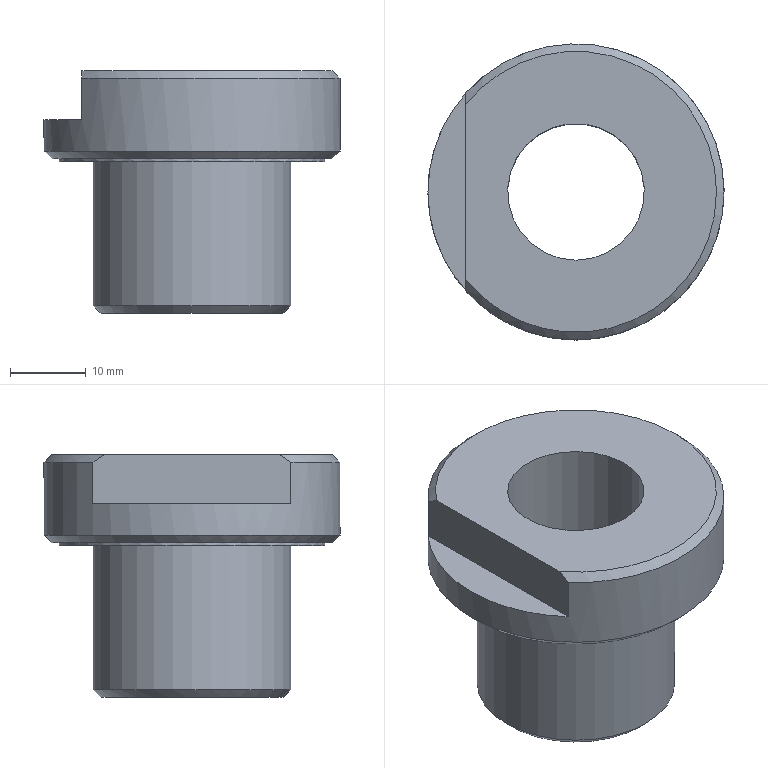Component | NX | REPL_DRILL_BUSH | 1 solid | 14 faces | box 39 x 39 x 32 mm | volume 15961 mm3 | plane 6 | cylinder 4 | cone 4 | commonest cylinder face diameters 26 x1 35 x1 39 x1 18 x1
STEP:
#1=CARTESIAN_POINT('',(0.,0.,0.));
#2=DIRECTION('',(0.,0.,1.));
#3=DIRECTION('',(1.,0.,0.));
#4=AXIS2_PLACEMENT_3D('',#1,#2,#3);
#5=CARTESIAN_POINT('',(32.,-10.,-160.));
#6=VERTEX_POINT('',#5);
#7=CARTESIAN_POINT('',(32.,-0.,-160.));
#8=DIRECTION('',(0.,0.,1.));
#9=DIRECTION('',(0.,-1.,0.));
#10=AXIS2_PLACEMENT_3D('',#7,#8,#9);
#11=CIRCLE('',#10,10.);
#12=CARTESIAN_POINT('',(32.,-0.,-160.));
#13=DIRECTION('',(0.,0.,-1.));
#14=DIRECTION('',(0.,-1.,0.));
#15=AXIS2_PLACEMENT_3D('',#12,#13,#14);
#16=PLANE('',#15);
#17=CARTESIAN_POINT('',(10.,0.));
#18=CARTESIAN_POINT('',(10.,-17.321));
#19=CARTESIAN_POINT('',(-5.,-8.66));
#20=CARTESIAN_POINT('',(-20.,-0.));
#21=CARTESIAN_POINT('',(-5.,8.66));
#22=CARTESIAN_POINT('',(10.,17.321));
#23=CARTESIAN_POINT('',(10.,0.));
#24=(BOUNDED_CURVE()B_SPLINE_CURVE(2,(#17,#18,#19,#20,#21,#22,#23),.UNSPECIFIED.,.T.,.F.)B_SPLINE_CURVE_WITH_KNOTS((1,2,2,2,2,1),(-2.094,0.,2.094,4.189,6.283,8.378),.UNSPECIFIED.)CURVE()GEOMETRIC_REPRESENTATION_ITEM()RATIONAL_B_SPLINE_CURVE((1.,0.5,1.,0.5,1.,0.5,1.))REPRESENTATION_ITEM(''));
#25=(GEOMETRIC_REPRESENTATION_CONTEXT(2)PARAMETRIC_REPRESENTATION_CONTEXT()REPRESENTATION_CONTEXT('',''));
#26=DEFINITIONAL_REPRESENTATION('',(#24),#25);
#27=PCURVE('',#16,#26);
#28=CARTESIAN_POINT('',(32.,-0.,-159.));
#29=DIRECTION('',(0.,0.,-1.));
#30=DIRECTION('',(0.,-1.,0.));
#31=AXIS2_PLACEMENT_3D('',#28,#29,#30);
#32=CONICAL_SURFACE('',#31,9.,0.7854);
#33=CARTESIAN_POINT('',(6.283,1.));
#34=DIRECTION('',(-1.,0.));
#35=VECTOR('',#34,1.);
#36=LINE('',#33,#35);
#37=(GEOMETRIC_REPRESENTATION_CONTEXT(2)PARAMETRIC_REPRESENTATION_CONTEXT()REPRESENTATION_CONTEXT('',''));
#38=DEFINITIONAL_REPRESENTATION('',(#36),#37);
#39=PCURVE('',#32,#38);
#40=SURFACE_CURVE('',#11,(#27,#39),.PCURVE_S1.);
#41=EDGE_CURVE('',#6,#6,#40,.T.);
#42=ORIENTED_EDGE('',*,*,#41,.T.);
#43=EDGE_LOOP('',(#42));
#44=FACE_BOUND('',#43,.T.);
#45=CARTESIAN_POINT('',(32.,-12.,-160.));
#46=VERTEX_POINT('',#45);
#47=CARTESIAN_POINT('',(32.,-0.,-160.));
#48=DIRECTION('',(0.,0.,-1.));
#49=DIRECTION('',(0.,-1.,0.));
#50=AXIS2_PLACEMENT_3D('',#47,#48,#49);
#51=CIRCLE('',#50,12.);
#52=CARTESIAN_POINT('',(0.,0.));
#53=DIRECTION('',(1.,0.));
#54=AXIS2_PLACEMENT_2D('',#52,#53);
#55=CIRCLE('',#54,12.);
#56=(GEOMETRIC_REPRESENTATION_CONTEXT(2)PARAMETRIC_REPRESENTATION_CONTEXT()REPRESENTATION_CONTEXT('',''));
#57=DEFINITIONAL_REPRESENTATION('',(#55),#56);
#58=PCURVE('',#16,#57);
#59=CARTESIAN_POINT('',(32.,-0.,-159.));
#60=DIRECTION('',(0.,0.,1.));
#61=DIRECTION('',(0.,1.,0.));
#62=AXIS2_PLACEMENT_3D('',#59,#60,#61);
#63=CONICAL_SURFACE('',#62,13.,0.7854);
#64=CARTESIAN_POINT('',(9.425,-1.));
#65=DIRECTION('',(-1.,0.));
#66=VECTOR('',#65,1.);
#67=LINE('',#64,#66);
#68=(GEOMETRIC_REPRESENTATION_CONTEXT(2)PARAMETRIC_REPRESENTATION_CONTEXT()REPRESENTATION_CONTEXT('',''));
#69=DEFINITIONAL_REPRESENTATION('',(#67),#68);
#70=PCURVE('',#63,#69);
#71=SURFACE_CURVE('',#51,(#58,#70),.PCURVE_S1.);
#72=EDGE_CURVE('',#46,#46,#71,.T.);
#73=ORIENTED_EDGE('',*,*,#72,.T.);
#74=EDGE_LOOP('',(#73));
#75=FACE_BOUND('',#74,.T.);
#76=ADVANCED_FACE('',(#44,#75),#16,.T.);
#77=CARTESIAN_POINT('',(32.,-13.,-159.));
#78=VERTEX_POINT('',#77);
#79=CARTESIAN_POINT('',(32.,-0.,-159.));
#80=DIRECTION('',(0.,0.,1.));
#81=DIRECTION('',(0.,-1.,0.));
#82=AXIS2_PLACEMENT_3D('',#79,#80,#81);
#83=CIRCLE('',#82,13.);
#84=CARTESIAN_POINT('',(32.,-0.,-160.));
#85=DIRECTION('',(0.,0.,1.));
#86=DIRECTION('',(0.,1.,0.));
#87=AXIS2_PLACEMENT_3D('',#84,#85,#86);
#88=CYLINDRICAL_SURFACE('',#87,13.);
#89=CARTESIAN_POINT('',(3.142,1.));
#90=DIRECTION('',(1.,0.));
#91=VECTOR('',#90,1.);
#92=LINE('',#89,#91);
#93=(GEOMETRIC_REPRESENTATION_CONTEXT(2)PARAMETRIC_REPRESENTATION_CONTEXT()REPRESENTATION_CONTEXT('',''));
#94=DEFINITIONAL_REPRESENTATION('',(#92),#93);
#95=PCURVE('',#88,#94);
#96=CARTESIAN_POINT('',(3.142,0.));
#97=DIRECTION('',(1.,0.));
#98=VECTOR('',#97,1.);
#99=LINE('',#96,#98);
#100=(GEOMETRIC_REPRESENTATION_CONTEXT(2)PARAMETRIC_REPRESENTATION_CONTEXT()REPRESENTATION_CONTEXT('',''));
#101=DEFINITIONAL_REPRESENTATION('',(#99),#100);
#102=PCURVE('',#63,#101);
#103=SURFACE_CURVE('',#83,(#95,#102),.PCURVE_S1.);
#104=EDGE_CURVE('',#78,#78,#103,.T.);
#105=ORIENTED_EDGE('',*,*,#104,.T.);
#106=CARTESIAN_POINT('',(32.,-13.,-140.));
#107=VERTEX_POINT('',#106);
#108=CARTESIAN_POINT('',(32.,-13.,-159.));
#109=CARTESIAN_POINT('',(32.,-13.,-140.));
#110=B_SPLINE_CURVE_WITH_KNOTS('',1,(#108,#109),.UNSPECIFIED.,.F.,.F.,(2,2),(1.,20.),.PIECEWISE_BEZIER_KNOTS.);
#111=CARTESIAN_POINT('',(9.425,0.));
#112=DIRECTION('',(0.,1.));
#113=VECTOR('',#112,1.);
#114=LINE('',#111,#113);
#115=(GEOMETRIC_REPRESENTATION_CONTEXT(2)PARAMETRIC_REPRESENTATION_CONTEXT()REPRESENTATION_CONTEXT('',''));
#116=DEFINITIONAL_REPRESENTATION('',(#114),#115);
#117=PCURVE('',#88,#116);
#118=CARTESIAN_POINT('',(3.142,0.));
#119=DIRECTION('',(0.,1.));
#120=VECTOR('',#119,1.);
#121=LINE('',#118,#120);
#122=(GEOMETRIC_REPRESENTATION_CONTEXT(2)PARAMETRIC_REPRESENTATION_CONTEXT()REPRESENTATION_CONTEXT('',''));
#123=DEFINITIONAL_REPRESENTATION('',(#121),#122);
#124=PCURVE('',#88,#123);
#125=SEAM_CURVE('',#110,(#117,#124),.PCURVE_S1.);
#126=EDGE_CURVE('',#78,#107,#125,.T.);
#127=ORIENTED_EDGE('',*,*,#126,.T.);
#128=CARTESIAN_POINT('',(32.,-0.,-140.));
#129=DIRECTION('',(0.,0.,1.));
#130=DIRECTION('',(0.,-1.,0.));
#131=AXIS2_PLACEMENT_3D('',#128,#129,#130);
#132=CIRCLE('',#131,13.);
#133=CARTESIAN_POINT('',(3.142,20.));
#134=DIRECTION('',(1.,0.));
#135=VECTOR('',#134,1.);
#136=LINE('',#133,#135);
#137=(GEOMETRIC_REPRESENTATION_CONTEXT(2)PARAMETRIC_REPRESENTATION_CONTEXT()REPRESENTATION_CONTEXT('',''));
#138=DEFINITIONAL_REPRESENTATION('',(#136),#137);
#139=PCURVE('',#88,#138);
#140=CARTESIAN_POINT('',(32.,-0.,-140.));
#141=DIRECTION('',(0.,0.,-1.));
#142=DIRECTION('',(0.,-1.,0.));
#143=AXIS2_PLACEMENT_3D('',#140,#141,#142);
#144=PLANE('',#143);
#145=CARTESIAN_POINT('',(13.,0.));
#146=CARTESIAN_POINT('',(13.,-22.517));
#147=CARTESIAN_POINT('',(-6.5,-11.258));
#148=CARTESIAN_POINT('',(-26.,-0.));
#149=CARTESIAN_POINT('',(-6.5,11.258));
#150=CARTESIAN_POINT('',(13.,22.517));
#151=CARTESIAN_POINT('',(13.,0.));
#152=(BOUNDED_CURVE()B_SPLINE_CURVE(2,(#145,#146,#147,#148,#149,#150,#151),.UNSPECIFIED.,.T.,.F.)B_SPLINE_CURVE_WITH_KNOTS((1,2,2,2,2,1),(-2.094,0.,2.094,4.189,6.283,8.378),.UNSPECIFIED.)CURVE()GEOMETRIC_REPRESENTATION_ITEM()RATIONAL_B_SPLINE_CURVE((1.,0.5,1.,0.5,1.,0.5,1.))REPRESENTATION_ITEM(''));
#153=(GEOMETRIC_REPRESENTATION_CONTEXT(2)PARAMETRIC_REPRESENTATION_CONTEXT()REPRESENTATION_CONTEXT('',''));
#154=DEFINITIONAL_REPRESENTATION('',(#152),#153);
#155=PCURVE('',#144,#154);
#156=SURFACE_CURVE('',#132,(#139,#155),.PCURVE_S1.);
#157=EDGE_CURVE('',#107,#107,#156,.T.);
#158=ORIENTED_EDGE('',*,*,#157,.F.);
#159=ORIENTED_EDGE('',*,*,#126,.F.);
#160=EDGE_LOOP('',(#105,#127,#158,#159));
#161=FACE_BOUND('',#160,.T.);
#162=ADVANCED_FACE('',(#161),#88,.T.);
#163=ORIENTED_EDGE('',*,*,#157,.T.);
#164=EDGE_LOOP('',(#163));
#165=FACE_BOUND('',#164,.T.);
#166=CARTESIAN_POINT('',(32.,17.5,-140.));
#167=VERTEX_POINT('',#166);
#168=CARTESIAN_POINT('',(32.,-0.,-140.));
#169=DIRECTION('',(0.,0.,1.));
#170=DIRECTION('',(0.,1.,0.));
#171=AXIS2_PLACEMENT_3D('',#168,#169,#170);
#172=CIRCLE('',#171,17.5);
#173=CARTESIAN_POINT('',(-17.5,0.));
#174=CARTESIAN_POINT('',(-17.5,30.311));
#175=CARTESIAN_POINT('',(8.75,15.155));
#176=CARTESIAN_POINT('',(35.,0.));
#177=CARTESIAN_POINT('',(8.75,-15.155));
#178=CARTESIAN_POINT('',(-17.5,-30.311));
#179=CARTESIAN_POINT('',(-17.5,0.));
#180=(BOUNDED_CURVE()B_SPLINE_CURVE(2,(#173,#174,#175,#176,#177,#178,#179),.UNSPECIFIED.,.T.,.F.)B_SPLINE_CURVE_WITH_KNOTS((1,2,2,2,2,1),(-2.094,0.,2.094,4.189,6.283,8.378),.UNSPECIFIED.)CURVE()GEOMETRIC_REPRESENTATION_ITEM()RATIONAL_B_SPLINE_CURVE((1.,0.5,1.,0.5,1.,0.5,1.))REPRESENTATION_ITEM(''));
#181=(GEOMETRIC_REPRESENTATION_CONTEXT(2)PARAMETRIC_REPRESENTATION_CONTEXT()REPRESENTATION_CONTEXT('',''));
#182=DEFINITIONAL_REPRESENTATION('',(#180),#181);
#183=PCURVE('',#144,#182);
#184=CARTESIAN_POINT('',(32.,-0.,-140.));
#185=DIRECTION('',(0.,0.,1.));
#186=DIRECTION('',(0.,1.,0.));
#187=AXIS2_PLACEMENT_3D('',#184,#185,#186);
#188=CYLINDRICAL_SURFACE('',#187,17.5);
#189=CARTESIAN_POINT('',(0.,0.));
#190=DIRECTION('',(1.,0.));
#191=VECTOR('',#190,1.);
#192=LINE('',#189,#191);
#193=(GEOMETRIC_REPRESENTATION_CONTEXT(2)PARAMETRIC_REPRESENTATION_CONTEXT()REPRESENTATION_CONTEXT('',''));
#194=DEFINITIONAL_REPRESENTATION('',(#192),#193);
#195=PCURVE('',#188,#194);
#196=SURFACE_CURVE('',#172,(#183,#195),.PCURVE_S1.);
#197=EDGE_CURVE('',#167,#167,#196,.T.);
#198=ORIENTED_EDGE('',*,*,#197,.F.);
#199=EDGE_LOOP('',(#198));
#200=FACE_BOUND('',#199,.T.);
#201=ADVANCED_FACE('',(#165,#200),#144,.T.);
#202=CARTESIAN_POINT('',(32.,17.5,-139.6));
#203=VERTEX_POINT('',#202);
#204=CARTESIAN_POINT('',(32.,-17.5,-139.6));
#205=VERTEX_POINT('',#204);
#206=CARTESIAN_POINT('',(32.,-0.,-139.6));
#207=DIRECTION('',(0.,0.,1.));
#208=DIRECTION('',(0.,-1.,0.));
#209=AXIS2_PLACEMENT_3D('',#206,#207,#208);
#210=CIRCLE('',#209,17.5);
#211=CARTESIAN_POINT('',(-3.142,0.4));
#212=DIRECTION('',(1.,0.));
#213=VECTOR('',#212,1.);
#214=LINE('',#211,#213);
#215=(GEOMETRIC_REPRESENTATION_CONTEXT(2)PARAMETRIC_REPRESENTATION_CONTEXT()REPRESENTATION_CONTEXT('',''));
#216=DEFINITIONAL_REPRESENTATION('',(#214),#215);
#217=PCURVE('',#188,#216);
#218=CARTESIAN_POINT('',(32.,-0.,-139.6));
#219=DIRECTION('',(0.,0.,-1.));
#220=DIRECTION('',(0.,-1.,0.));
#221=AXIS2_PLACEMENT_3D('',#218,#219,#220);
#222=PLANE('',#221);
#223=CARTESIAN_POINT('',(17.5,0.));
#224=CARTESIAN_POINT('',(17.5,-30.311));
#225=CARTESIAN_POINT('',(-8.75,-15.155));
#226=CARTESIAN_POINT('',(-35.,-0.));
#227=CARTESIAN_POINT('',(-8.75,15.155));
#228=CARTESIAN_POINT('',(17.5,30.311));
#229=CARTESIAN_POINT('',(17.5,0.));
#230=(BOUNDED_CURVE()B_SPLINE_CURVE(2,(#223,#224,#225,#226,#227,#228,#229),.UNSPECIFIED.,.T.,.F.)B_SPLINE_CURVE_WITH_KNOTS((1,2,2,2,2,1),(-2.094,0.,2.094,4.189,6.283,8.378),.UNSPECIFIED.)CURVE()GEOMETRIC_REPRESENTATION_ITEM()RATIONAL_B_SPLINE_CURVE((1.,0.5,1.,0.5,1.,0.5,1.))REPRESENTATION_ITEM(''));
#231=(GEOMETRIC_REPRESENTATION_CONTEXT(2)PARAMETRIC_REPRESENTATION_CONTEXT()REPRESENTATION_CONTEXT('',''));
#232=DEFINITIONAL_REPRESENTATION('',(#230),#231);
#233=PCURVE('',#222,#232);
#234=SURFACE_CURVE('',#210,(#217,#233),.PCURVE_S1.);
#235=EDGE_CURVE('',#203,#205,#234,.T.);
#236=ORIENTED_EDGE('',*,*,#235,.F.);
#237=CARTESIAN_POINT('',(32.,17.5,-140.));
#238=CARTESIAN_POINT('',(32.,17.5,-139.6));
#239=B_SPLINE_CURVE_WITH_KNOTS('',1,(#237,#238),.UNSPECIFIED.,.F.,.F.,(2,2),(0.,0.4),.PIECEWISE_BEZIER_KNOTS.);
#240=CARTESIAN_POINT('',(0.,0.));
#241=DIRECTION('',(0.,1.));
#242=VECTOR('',#241,1.);
#243=LINE('',#240,#242);
#244=(GEOMETRIC_REPRESENTATION_CONTEXT(2)PARAMETRIC_REPRESENTATION_CONTEXT()REPRESENTATION_CONTEXT('',''));
#245=DEFINITIONAL_REPRESENTATION('',(#243),#244);
#246=PCURVE('',#188,#245);
#247=CARTESIAN_POINT('',(6.283,0.));
#248=DIRECTION('',(0.,1.));
#249=VECTOR('',#248,1.);
#250=LINE('',#247,#249);
#251=(GEOMETRIC_REPRESENTATION_CONTEXT(2)PARAMETRIC_REPRESENTATION_CONTEXT()REPRESENTATION_CONTEXT('',''));
#252=DEFINITIONAL_REPRESENTATION('',(#250),#251);
#253=PCURVE('',#188,#252);
#254=SEAM_CURVE('',#239,(#246,#253),.PCURVE_S1.);
#255=EDGE_CURVE('',#167,#203,#254,.T.);
#256=ORIENTED_EDGE('',*,*,#255,.F.);
#257=ORIENTED_EDGE('',*,*,#197,.T.);
#258=ORIENTED_EDGE('',*,*,#255,.T.);
#259=CARTESIAN_POINT('',(32.,-0.,-139.6));
#260=DIRECTION('',(0.,0.,1.));
#261=DIRECTION('',(0.,-1.,0.));
#262=AXIS2_PLACEMENT_3D('',#259,#260,#261);
#263=CIRCLE('',#262,17.5);
#264=CARTESIAN_POINT('',(3.142,0.4));
#265=DIRECTION('',(1.,0.));
#266=VECTOR('',#265,1.);
#267=LINE('',#264,#266);
#268=(GEOMETRIC_REPRESENTATION_CONTEXT(2)PARAMETRIC_REPRESENTATION_CONTEXT()REPRESENTATION_CONTEXT('',''));
#269=DEFINITIONAL_REPRESENTATION('',(#267),#268);
#270=PCURVE('',#188,#269);
#271=CARTESIAN_POINT('',(17.5,0.));
#272=CARTESIAN_POINT('',(17.5,-30.311));
#273=CARTESIAN_POINT('',(-8.75,-15.155));
#274=CARTESIAN_POINT('',(-35.,-0.));
#275=CARTESIAN_POINT('',(-8.75,15.155));
#276=CARTESIAN_POINT('',(17.5,30.311));
#277=CARTESIAN_POINT('',(17.5,0.));
#278=(BOUNDED_CURVE()B_SPLINE_CURVE(2,(#271,#272,#273,#274,#275,#276,#277),.UNSPECIFIED.,.T.,.F.)B_SPLINE_CURVE_WITH_KNOTS((1,2,2,2,2,1),(-2.094,0.,2.094,4.189,6.283,8.378),.UNSPECIFIED.)CURVE()GEOMETRIC_REPRESENTATION_ITEM()RATIONAL_B_SPLINE_CURVE((1.,0.5,1.,0.5,1.,0.5,1.))REPRESENTATION_ITEM(''));
#279=(GEOMETRIC_REPRESENTATION_CONTEXT(2)PARAMETRIC_REPRESENTATION_CONTEXT()REPRESENTATION_CONTEXT('',''));
#280=DEFINITIONAL_REPRESENTATION('',(#278),#279);
#281=PCURVE('',#222,#280);
#282=SURFACE_CURVE('',#263,(#270,#281),.PCURVE_S1.);
#283=EDGE_CURVE('',#205,#203,#282,.T.);
#284=ORIENTED_EDGE('',*,*,#283,.F.);
#285=EDGE_LOOP('',(#236,#256,#257,#258,#284));
#286=FACE_BOUND('',#285,.T.);
#287=ADVANCED_FACE('',(#286),#188,.T.);
#288=CARTESIAN_POINT('',(32.,-9.,-128.));
#289=VERTEX_POINT('',#288);
#290=CARTESIAN_POINT('',(32.,-0.,-128.));
#291=DIRECTION('',(0.,0.,-1.));
#292=DIRECTION('',(0.,-1.,0.));
#293=AXIS2_PLACEMENT_3D('',#290,#291,#292);
#294=CIRCLE('',#293,9.);
#295=CARTESIAN_POINT('',(32.,-0.,-128.));
#296=DIRECTION('',(0.,0.,1.));
#297=DIRECTION('',(0.,1.,0.));
#298=AXIS2_PLACEMENT_3D('',#295,#296,#297);
#299=PLANE('',#298);
#300=CARTESIAN_POINT('',(-9.,0.));
#301=CARTESIAN_POINT('',(-9.,15.588));
#302=CARTESIAN_POINT('',(4.5,7.794));
#303=CARTESIAN_POINT('',(18.,0.));
#304=CARTESIAN_POINT('',(4.5,-7.794));
#305=CARTESIAN_POINT('',(-9.,-15.588));
#306=CARTESIAN_POINT('',(-9.,0.));
#307=(BOUNDED_CURVE()B_SPLINE_CURVE(2,(#300,#301,#302,#303,#304,#305,#306),.UNSPECIFIED.,.T.,.F.)B_SPLINE_CURVE_WITH_KNOTS((1,2,2,2,2,1),(-2.094,0.,2.094,4.189,6.283,8.378),.UNSPECIFIED.)CURVE()GEOMETRIC_REPRESENTATION_ITEM()RATIONAL_B_SPLINE_CURVE((1.,0.5,1.,0.5,1.,0.5,1.))REPRESENTATION_ITEM(''));
#308=(GEOMETRIC_REPRESENTATION_CONTEXT(2)PARAMETRIC_REPRESENTATION_CONTEXT()REPRESENTATION_CONTEXT('',''));
#309=DEFINITIONAL_REPRESENTATION('',(#307),#308);
#310=PCURVE('',#299,#309);
#311=CARTESIAN_POINT('',(32.,-0.,-128.));
#312=DIRECTION('',(0.,0.,-1.));
#313=DIRECTION('',(0.,-1.,0.));
#314=AXIS2_PLACEMENT_3D('',#311,#312,#313);
#315=CYLINDRICAL_SURFACE('',#314,9.);
#316=CARTESIAN_POINT('',(0.,0.));
#317=DIRECTION('',(1.,0.));
#318=VECTOR('',#317,1.);
#319=LINE('',#316,#318);
#320=(GEOMETRIC_REPRESENTATION_CONTEXT(2)PARAMETRIC_REPRESENTATION_CONTEXT()REPRESENTATION_CONTEXT('',''));
#321=DEFINITIONAL_REPRESENTATION('',(#319),#320);
#322=PCURVE('',#315,#321);
#323=SURFACE_CURVE('',#294,(#310,#322),.PCURVE_S1.);
#324=EDGE_CURVE('',#289,#289,#323,.T.);
#325=ORIENTED_EDGE('',*,*,#324,.T.);
#326=EDGE_LOOP('',(#325));
#327=FACE_BOUND('',#326,.T.);
#328=CARTESIAN_POINT('',(17.5,-11.489,-128.));
#329=VERTEX_POINT('',#328);
#330=CARTESIAN_POINT('',(17.5,11.489,-128.));
#331=VERTEX_POINT('',#330);
#332=CARTESIAN_POINT('',(17.5,-34.5,-128.));
#333=DIRECTION('',(-0.,1.,0.));
#334=VECTOR('',#333,1.);
#335=LINE('',#332,#334);
#336=CARTESIAN_POINT('',(-34.5,14.5));
#337=DIRECTION('',(1.,0.));
#338=VECTOR('',#337,1.);
#339=LINE('',#336,#338);
#340=(GEOMETRIC_REPRESENTATION_CONTEXT(2)PARAMETRIC_REPRESENTATION_CONTEXT()REPRESENTATION_CONTEXT('',''));
#341=DEFINITIONAL_REPRESENTATION('',(#339),#340);
#342=PCURVE('',#299,#341);
#343=CARTESIAN_POINT('',(17.5,-34.5,-134.5));
#344=DIRECTION('',(1.,0.,0.));
#345=DIRECTION('',(-0.,1.,0.));
#346=AXIS2_PLACEMENT_3D('',#343,#344,#345);
#347=PLANE('',#346);
#348=CARTESIAN_POINT('',(0.,6.5));
#349=DIRECTION('',(1.,0.));
#350=VECTOR('',#349,1.);
#351=LINE('',#348,#350);
#352=(GEOMETRIC_REPRESENTATION_CONTEXT(2)PARAMETRIC_REPRESENTATION_CONTEXT()REPRESENTATION_CONTEXT('',''));
#353=DEFINITIONAL_REPRESENTATION('',(#351),#352);
#354=PCURVE('',#347,#353);
#355=SURFACE_CURVE('',#335,(#342,#354),.PCURVE_S1.);
#356=EDGE_CURVE('',#329,#331,#355,.T.);
#357=ORIENTED_EDGE('',*,*,#356,.F.);
#358=CARTESIAN_POINT('',(32.,-0.,-128.));
#359=DIRECTION('',(0.,0.,1.));
#360=DIRECTION('',(0.,1.,0.));
#361=AXIS2_PLACEMENT_3D('',#358,#359,#360);
#362=CIRCLE('',#361,18.5);
#363=CARTESIAN_POINT('',(0.,0.));
#364=DIRECTION('',(1.,0.));
#365=AXIS2_PLACEMENT_2D('',#363,#364);
#366=CIRCLE('',#365,18.5);
#367=(GEOMETRIC_REPRESENTATION_CONTEXT(2)PARAMETRIC_REPRESENTATION_CONTEXT()REPRESENTATION_CONTEXT('',''));
#368=DEFINITIONAL_REPRESENTATION('',(#366),#367);
#369=PCURVE('',#299,#368);
#370=CARTESIAN_POINT('',(32.,-0.,-129.));
#371=DIRECTION('',(0.,0.,-1.));
#372=DIRECTION('',(0.,-1.,0.));
#373=AXIS2_PLACEMENT_3D('',#370,#371,#372);
#374=CONICAL_SURFACE('',#373,19.5,0.7854);
#375=CARTESIAN_POINT('',(9.425,-1.));
#376=DIRECTION('',(-1.,-0.));
#377=VECTOR('',#376,1.);
#378=LINE('',#375,#377);
#379=(GEOMETRIC_REPRESENTATION_CONTEXT(2)PARAMETRIC_REPRESENTATION_CONTEXT()REPRESENTATION_CONTEXT('',''));
#380=DEFINITIONAL_REPRESENTATION('',(#378),#379);
#381=PCURVE('',#374,#380);
#382=SURFACE_CURVE('',#362,(#369,#381),.PCURVE_S1.);
#383=EDGE_CURVE('',#329,#331,#382,.T.);
#384=ORIENTED_EDGE('',*,*,#383,.T.);
#385=EDGE_LOOP('',(#357,#384));
#386=FACE_BOUND('',#385,.T.);
#387=ADVANCED_FACE('',(#327,#386),#299,.T.);
#388=CARTESIAN_POINT('',(32.,-18.5,-139.6));
#389=VERTEX_POINT('',#388);
#390=CARTESIAN_POINT('',(32.,-0.,-139.6));
#391=DIRECTION('',(0.,0.,-1.));
#392=DIRECTION('',(0.,-1.,0.));
#393=AXIS2_PLACEMENT_3D('',#390,#391,#392);
#394=CIRCLE('',#393,18.5);
#395=CARTESIAN_POINT('',(0.,0.));
#396=DIRECTION('',(1.,0.));
#397=AXIS2_PLACEMENT_2D('',#395,#396);
#398=CIRCLE('',#397,18.5);
#399=(GEOMETRIC_REPRESENTATION_CONTEXT(2)PARAMETRIC_REPRESENTATION_CONTEXT()REPRESENTATION_CONTEXT('',''));
#400=DEFINITIONAL_REPRESENTATION('',(#398),#399);
#401=PCURVE('',#222,#400);
#402=CARTESIAN_POINT('',(32.,-0.,-138.6));
#403=DIRECTION('',(0.,0.,1.));
#404=DIRECTION('',(0.,1.,0.));
#405=AXIS2_PLACEMENT_3D('',#402,#403,#404);
#406=CONICAL_SURFACE('',#405,19.5,0.7854);
#407=CARTESIAN_POINT('',(9.425,-1.));
#408=DIRECTION('',(-1.,0.));
#409=VECTOR('',#408,1.);
#410=LINE('',#407,#409);
#411=(GEOMETRIC_REPRESENTATION_CONTEXT(2)PARAMETRIC_REPRESENTATION_CONTEXT()REPRESENTATION_CONTEXT('',''));
#412=DEFINITIONAL_REPRESENTATION('',(#410),#411);
#413=PCURVE('',#406,#412);
#414=SURFACE_CURVE('',#394,(#401,#413),.PCURVE_S1.);
#415=EDGE_CURVE('',#389,#389,#414,.T.);
#416=ORIENTED_EDGE('',*,*,#415,.T.);
#417=EDGE_LOOP('',(#416));
#418=FACE_BOUND('',#417,.T.);
#419=ORIENTED_EDGE('',*,*,#283,.T.);
#420=ORIENTED_EDGE('',*,*,#235,.T.);
#421=EDGE_LOOP('',(#419,#420));
#422=FACE_BOUND('',#421,.T.);
#423=ADVANCED_FACE('',(#418,#422),#222,.T.);
#424=CARTESIAN_POINT('',(32.,-19.5,-138.6));
#425=VERTEX_POINT('',#424);
#426=CARTESIAN_POINT('',(17.5,13.038,-138.6));
#427=VERTEX_POINT('',#426);
#428=CARTESIAN_POINT('',(32.,-0.,-138.6));
#429=DIRECTION('',(0.,0.,1.));
#430=DIRECTION('',(0.,-1.,0.));
#431=AXIS2_PLACEMENT_3D('',#428,#429,#430);
#432=CIRCLE('',#431,19.5);
#433=CARTESIAN_POINT('',(32.,-0.,-139.6));
#434=DIRECTION('',(0.,0.,1.));
#435=DIRECTION('',(0.,1.,0.));
#436=AXIS2_PLACEMENT_3D('',#433,#434,#435);
#437=CYLINDRICAL_SURFACE('',#436,19.5);
#438=CARTESIAN_POINT('',(3.142,1.));
#439=DIRECTION('',(1.,0.));
#440=VECTOR('',#439,1.);
#441=LINE('',#438,#440);
#442=(GEOMETRIC_REPRESENTATION_CONTEXT(2)PARAMETRIC_REPRESENTATION_CONTEXT()REPRESENTATION_CONTEXT('',''));
#443=DEFINITIONAL_REPRESENTATION('',(#441),#442);
#444=PCURVE('',#437,#443);
#445=CARTESIAN_POINT('',(3.142,0.));
#446=DIRECTION('',(1.,0.));
#447=VECTOR('',#446,1.);
#448=LINE('',#445,#447);
#449=(GEOMETRIC_REPRESENTATION_CONTEXT(2)PARAMETRIC_REPRESENTATION_CONTEXT()REPRESENTATION_CONTEXT('',''));
#450=DEFINITIONAL_REPRESENTATION('',(#448),#449);
#451=PCURVE('',#406,#450);
#452=SURFACE_CURVE('',#432,(#444,#451),.PCURVE_S1.);
#453=EDGE_CURVE('',#425,#427,#452,.T.);
#454=ORIENTED_EDGE('',*,*,#453,.T.);
#455=CARTESIAN_POINT('',(17.5,13.038,-134.5));
#456=VERTEX_POINT('',#455);
#457=CARTESIAN_POINT('',(17.5,13.038,-138.6));
#458=CARTESIAN_POINT('',(17.5,13.038,-134.5));
#459=B_SPLINE_CURVE_WITH_KNOTS('',1,(#457,#458),.UNSPECIFIED.,.F.,.F.,(2,2),(1.,5.1),.PIECEWISE_BEZIER_KNOTS.);
#460=CARTESIAN_POINT('',(7.122,0.));
#461=DIRECTION('',(0.,1.));
#462=VECTOR('',#461,1.);
#463=LINE('',#460,#462);
#464=(GEOMETRIC_REPRESENTATION_CONTEXT(2)PARAMETRIC_REPRESENTATION_CONTEXT()REPRESENTATION_CONTEXT('',''));
#465=DEFINITIONAL_REPRESENTATION('',(#463),#464);
#466=PCURVE('',#437,#465);
#467=CARTESIAN_POINT('',(0.8384,0.));
#468=DIRECTION('',(0.,1.));
#469=VECTOR('',#468,1.);
#470=LINE('',#467,#469);
#471=(GEOMETRIC_REPRESENTATION_CONTEXT(2)PARAMETRIC_REPRESENTATION_CONTEXT()REPRESENTATION_CONTEXT('',''));
#472=DEFINITIONAL_REPRESENTATION('',(#470),#471);
#473=PCURVE('',#437,#472);
#474=SEAM_CURVE('',#459,(#466,#473),.PCURVE_S1.);
#475=EDGE_CURVE('',#427,#456,#474,.T.);
#476=ORIENTED_EDGE('',*,*,#475,.T.);
#477=CARTESIAN_POINT('',(17.5,13.038,-129.));
#478=VERTEX_POINT('',#477);
#479=CARTESIAN_POINT('',(17.5,13.038,-139.6));
#480=DIRECTION('',(0.,0.,-1.));
#481=VECTOR('',#480,1.);
#482=LINE('',#479,#481);
#483=CARTESIAN_POINT('',(7.122,0.));
#484=DIRECTION('',(0.,-1.));
#485=VECTOR('',#484,1.);
#486=LINE('',#483,#485);
#487=(GEOMETRIC_REPRESENTATION_CONTEXT(2)PARAMETRIC_REPRESENTATION_CONTEXT()REPRESENTATION_CONTEXT('',''));
#488=DEFINITIONAL_REPRESENTATION('',(#486),#487);
#489=PCURVE('',#437,#488);
#490=CARTESIAN_POINT('',(47.538,-5.1));
#491=DIRECTION('',(0.,-1.));
#492=VECTOR('',#491,1.);
#493=LINE('',#490,#492);
#494=(GEOMETRIC_REPRESENTATION_CONTEXT(2)PARAMETRIC_REPRESENTATION_CONTEXT()REPRESENTATION_CONTEXT('',''));
#495=DEFINITIONAL_REPRESENTATION('',(#493),#494);
#496=PCURVE('',#347,#495);
#497=SURFACE_CURVE('',#482,(#489,#496),.PCURVE_S1.);
#498=EDGE_CURVE('',#478,#456,#497,.T.);
#499=ORIENTED_EDGE('',*,*,#498,.F.);
#500=CARTESIAN_POINT('',(17.5,-13.038,-129.));
#501=VERTEX_POINT('',#500);
#502=CARTESIAN_POINT('',(32.,-0.,-129.));
#503=DIRECTION('',(0.,0.,-1.));
#504=DIRECTION('',(0.,1.,0.));
#505=AXIS2_PLACEMENT_3D('',#502,#503,#504);
#506=CIRCLE('',#505,19.5);
#507=CARTESIAN_POINT('',(12.566,10.6));
#508=DIRECTION('',(-1.,0.));
#509=VECTOR('',#508,1.);
#510=LINE('',#507,#509);
#511=(GEOMETRIC_REPRESENTATION_CONTEXT(2)PARAMETRIC_REPRESENTATION_CONTEXT()REPRESENTATION_CONTEXT('',''));
#512=DEFINITIONAL_REPRESENTATION('',(#510),#511);
#513=PCURVE('',#437,#512);
#514=CARTESIAN_POINT('',(-3.142,0.));
#515=DIRECTION('',(1.,0.));
#516=VECTOR('',#515,1.);
#517=LINE('',#514,#516);
#518=(GEOMETRIC_REPRESENTATION_CONTEXT(2)PARAMETRIC_REPRESENTATION_CONTEXT()REPRESENTATION_CONTEXT('',''));
#519=DEFINITIONAL_REPRESENTATION('',(#517),#518);
#520=PCURVE('',#374,#519);
#521=SURFACE_CURVE('',#506,(#513,#520),.PCURVE_S1.);
#522=EDGE_CURVE('',#478,#501,#521,.T.);
#523=ORIENTED_EDGE('',*,*,#522,.T.);
#524=CARTESIAN_POINT('',(17.5,-13.038,-134.5));
#525=VERTEX_POINT('',#524);
#526=CARTESIAN_POINT('',(17.5,-13.038,-139.6));
#527=DIRECTION('',(0.,0.,1.));
#528=VECTOR('',#527,1.);
#529=LINE('',#526,#528);
#530=CARTESIAN_POINT('',(2.303,0.));
#531=DIRECTION('',(0.,1.));
#532=VECTOR('',#531,1.);
#533=LINE('',#530,#532);
#534=(GEOMETRIC_REPRESENTATION_CONTEXT(2)PARAMETRIC_REPRESENTATION_CONTEXT()REPRESENTATION_CONTEXT('',''));
#535=DEFINITIONAL_REPRESENTATION('',(#533),#534);
#536=PCURVE('',#437,#535);
#537=CARTESIAN_POINT('',(21.462,-5.1));
#538=DIRECTION('',(0.,1.));
#539=VECTOR('',#538,1.);
#540=LINE('',#537,#539);
#541=(GEOMETRIC_REPRESENTATION_CONTEXT(2)PARAMETRIC_REPRESENTATION_CONTEXT()REPRESENTATION_CONTEXT('',''));
#542=DEFINITIONAL_REPRESENTATION('',(#540),#541);
#543=PCURVE('',#347,#542);
#544=SURFACE_CURVE('',#529,(#536,#543),.PCURVE_S1.);
#545=EDGE_CURVE('',#525,#501,#544,.T.);
#546=ORIENTED_EDGE('',*,*,#545,.F.);
#547=CARTESIAN_POINT('',(32.,-0.,-134.5));
#548=DIRECTION('',(0.,0.,-1.));
#549=DIRECTION('',(0.,1.,0.));
#550=AXIS2_PLACEMENT_3D('',#547,#548,#549);
#551=CIRCLE('',#550,19.5);
#552=CARTESIAN_POINT('',(6.283,5.1));
#553=DIRECTION('',(-1.,0.));
#554=VECTOR('',#553,1.);
#555=LINE('',#552,#554);
#556=(GEOMETRIC_REPRESENTATION_CONTEXT(2)PARAMETRIC_REPRESENTATION_CONTEXT()REPRESENTATION_CONTEXT('',''));
#557=DEFINITIONAL_REPRESENTATION('',(#555),#556);
#558=PCURVE('',#437,#557);
#559=CARTESIAN_POINT('',(32.,-0.,-134.5));
#560=DIRECTION('',(0.,0.,1.));
#561=DIRECTION('',(0.,1.,0.));
#562=AXIS2_PLACEMENT_3D('',#559,#560,#561);
#563=PLANE('',#562);
#564=CARTESIAN_POINT('',(19.5,0.));
#565=CARTESIAN_POINT('',(19.5,-33.775));
#566=CARTESIAN_POINT('',(-9.75,-16.887));
#567=CARTESIAN_POINT('',(-39.,-0.));
#568=CARTESIAN_POINT('',(-9.75,16.887));
#569=CARTESIAN_POINT('',(19.5,33.775));
#570=CARTESIAN_POINT('',(19.5,0.));
#571=(BOUNDED_CURVE()B_SPLINE_CURVE(2,(#564,#565,#566,#567,#568,#569,#570),.UNSPECIFIED.,.T.,.F.)B_SPLINE_CURVE_WITH_KNOTS((1,2,2,2,2,1),(-2.094,0.,2.094,4.189,6.283,8.378),.UNSPECIFIED.)CURVE()GEOMETRIC_REPRESENTATION_ITEM()RATIONAL_B_SPLINE_CURVE((1.,0.5,1.,0.5,1.,0.5,1.))REPRESENTATION_ITEM(''));
#572=(GEOMETRIC_REPRESENTATION_CONTEXT(2)PARAMETRIC_REPRESENTATION_CONTEXT()REPRESENTATION_CONTEXT('',''));
#573=DEFINITIONAL_REPRESENTATION('',(#571),#572);
#574=PCURVE('',#563,#573);
#575=SURFACE_CURVE('',#551,(#558,#574),.PCURVE_S1.);
#576=EDGE_CURVE('',#525,#456,#575,.T.);
#577=ORIENTED_EDGE('',*,*,#576,.T.);
#578=ORIENTED_EDGE('',*,*,#475,.F.);
#579=CARTESIAN_POINT('',(32.,-0.,-138.6));
#580=DIRECTION('',(0.,0.,1.));
#581=DIRECTION('',(0.,-1.,0.));
#582=AXIS2_PLACEMENT_3D('',#579,#580,#581);
#583=CIRCLE('',#582,19.5);
#584=CARTESIAN_POINT('',(-3.142,1.));
#585=DIRECTION('',(1.,0.));
#586=VECTOR('',#585,1.);
#587=LINE('',#584,#586);
#588=(GEOMETRIC_REPRESENTATION_CONTEXT(2)PARAMETRIC_REPRESENTATION_CONTEXT()REPRESENTATION_CONTEXT('',''));
#589=DEFINITIONAL_REPRESENTATION('',(#587),#588);
#590=PCURVE('',#437,#589);
#591=CARTESIAN_POINT('',(3.142,0.));
#592=DIRECTION('',(1.,0.));
#593=VECTOR('',#592,1.);
#594=LINE('',#591,#593);
#595=(GEOMETRIC_REPRESENTATION_CONTEXT(2)PARAMETRIC_REPRESENTATION_CONTEXT()REPRESENTATION_CONTEXT('',''));
#596=DEFINITIONAL_REPRESENTATION('',(#594),#595);
#597=PCURVE('',#406,#596);
#598=SURFACE_CURVE('',#583,(#590,#597),.PCURVE_S1.);
#599=EDGE_CURVE('',#427,#425,#598,.T.);
#600=ORIENTED_EDGE('',*,*,#599,.T.);
#601=EDGE_LOOP('',(#454,#476,#499,#523,#546,#577,#578,#600));
#602=FACE_BOUND('',#601,.T.);
#603=ADVANCED_FACE('',(#602),#437,.T.);
#604=ORIENTED_EDGE('',*,*,#545,.T.);
#605=CARTESIAN_POINT('',(17.5,-13.038,-129.));
#606=CARTESIAN_POINT('',(17.5,-12.527,-128.658));
#607=CARTESIAN_POINT('',(17.5,-12.011,-128.324));
#608=CARTESIAN_POINT('',(17.5,-11.489,-128.));
#609=B_SPLINE_CURVE_WITH_KNOTS('',3,(#605,#606,#607,#608),.UNSPECIFIED.,.F.,.F.,(4,4),(0.,1.),.PIECEWISE_BEZIER_KNOTS.);
#610=CARTESIAN_POINT('',(21.462,5.5));
#611=CARTESIAN_POINT('',(21.973,5.842));
#612=CARTESIAN_POINT('',(22.489,6.176));
#613=CARTESIAN_POINT('',(23.011,6.5));
#614=B_SPLINE_CURVE_WITH_KNOTS('',3,(#610,#611,#612,#613),.UNSPECIFIED.,.F.,.F.,(4,4),(0.,1.),.PIECEWISE_BEZIER_KNOTS.);
#615=(GEOMETRIC_REPRESENTATION_CONTEXT(2)PARAMETRIC_REPRESENTATION_CONTEXT()REPRESENTATION_CONTEXT('',''));
#616=DEFINITIONAL_REPRESENTATION('',(#614),#615);
#617=PCURVE('',#347,#616);
#618=CARTESIAN_POINT('',(7.122,-0.));
#619=CARTESIAN_POINT('',(7.184,-1.));
#620=B_SPLINE_CURVE_WITH_KNOTS('',1,(#618,#619),.UNSPECIFIED.,.F.,.F.,(2,2),(0.,1.),.PIECEWISE_BEZIER_KNOTS.);
#621=(GEOMETRIC_REPRESENTATION_CONTEXT(2)PARAMETRIC_REPRESENTATION_CONTEXT()REPRESENTATION_CONTEXT('',''));
#622=DEFINITIONAL_REPRESENTATION('',(#620),#621);
#623=PCURVE('',#374,#622);
#624=SURFACE_CURVE('',#609,(#617,#623),.PCURVE_S1.);
#625=EDGE_CURVE('',#501,#329,#624,.T.);
#626=ORIENTED_EDGE('',*,*,#625,.T.);
#627=ORIENTED_EDGE('',*,*,#356,.T.);
#628=CARTESIAN_POINT('',(17.5,11.489,-128.));
#629=CARTESIAN_POINT('',(17.5,12.011,-128.324));
#630=CARTESIAN_POINT('',(17.5,12.527,-128.658));
#631=CARTESIAN_POINT('',(17.5,13.038,-129.));
#632=B_SPLINE_CURVE_WITH_KNOTS('',3,(#628,#629,#630,#631),.UNSPECIFIED.,.F.,.F.,(4,4),(0.,1.),.PIECEWISE_BEZIER_KNOTS.);
#633=CARTESIAN_POINT('',(45.989,6.5));
#634=CARTESIAN_POINT('',(46.511,6.176));
#635=CARTESIAN_POINT('',(47.027,5.842));
#636=CARTESIAN_POINT('',(47.538,5.5));
#637=B_SPLINE_CURVE_WITH_KNOTS('',3,(#633,#634,#635,#636),.UNSPECIFIED.,.F.,.F.,(4,4),(0.,1.),.PIECEWISE_BEZIER_KNOTS.);
#638=(GEOMETRIC_REPRESENTATION_CONTEXT(2)PARAMETRIC_REPRESENTATION_CONTEXT()REPRESENTATION_CONTEXT('',''));
#639=DEFINITIONAL_REPRESENTATION('',(#637),#638);
#640=PCURVE('',#347,#639);
#641=CARTESIAN_POINT('',(2.241,-1.));
#642=CARTESIAN_POINT('',(2.303,-0.));
#643=B_SPLINE_CURVE_WITH_KNOTS('',1,(#641,#642),.UNSPECIFIED.,.F.,.F.,(2,2),(0.,1.),.PIECEWISE_BEZIER_KNOTS.);
#644=(GEOMETRIC_REPRESENTATION_CONTEXT(2)PARAMETRIC_REPRESENTATION_CONTEXT()REPRESENTATION_CONTEXT('',''));
#645=DEFINITIONAL_REPRESENTATION('',(#643),#644);
#646=PCURVE('',#374,#645);
#647=SURFACE_CURVE('',#632,(#640,#646),.PCURVE_S1.);
#648=EDGE_CURVE('',#331,#478,#647,.T.);
#649=ORIENTED_EDGE('',*,*,#648,.T.);
#650=ORIENTED_EDGE('',*,*,#498,.T.);
#651=CARTESIAN_POINT('',(17.5,-34.5,-134.5));
#652=DIRECTION('',(0.,-1.,0.));
#653=VECTOR('',#652,1.);
#654=LINE('',#651,#653);
#655=CARTESIAN_POINT('',(0.,0.));
#656=DIRECTION('',(-1.,0.));
#657=VECTOR('',#656,1.);
#658=LINE('',#655,#657);
#659=(GEOMETRIC_REPRESENTATION_CONTEXT(2)PARAMETRIC_REPRESENTATION_CONTEXT()REPRESENTATION_CONTEXT('',''));
#660=DEFINITIONAL_REPRESENTATION('',(#658),#659);
#661=PCURVE('',#347,#660);
#662=CARTESIAN_POINT('',(-34.5,14.5));
#663=DIRECTION('',(-1.,-0.));
#664=VECTOR('',#663,1.);
#665=LINE('',#662,#664);
#666=(GEOMETRIC_REPRESENTATION_CONTEXT(2)PARAMETRIC_REPRESENTATION_CONTEXT()REPRESENTATION_CONTEXT('',''));
#667=DEFINITIONAL_REPRESENTATION('',(#665),#666);
#668=PCURVE('',#563,#667);
#669=SURFACE_CURVE('',#654,(#661,#668),.PCURVE_S1.);
#670=EDGE_CURVE('',#456,#525,#669,.T.);
#671=ORIENTED_EDGE('',*,*,#670,.T.);
#672=EDGE_LOOP('',(#604,#626,#627,#649,#650,#671));
#673=FACE_BOUND('',#672,.T.);
#674=ADVANCED_FACE('',(#673),#347,.F.);
#675=ORIENTED_EDGE('',*,*,#670,.F.);
#676=ORIENTED_EDGE('',*,*,#576,.F.);
#677=EDGE_LOOP('',(#675,#676));
#678=FACE_BOUND('',#677,.T.);
#679=ADVANCED_FACE('',(#678),#563,.T.);
#680=CARTESIAN_POINT('',(32.,-9.,-159.));
#681=VERTEX_POINT('',#680);
#682=CARTESIAN_POINT('',(32.,-0.,-159.));
#683=DIRECTION('',(0.,0.,-1.));
#684=DIRECTION('',(0.,-1.,0.));
#685=AXIS2_PLACEMENT_3D('',#682,#683,#684);
#686=CIRCLE('',#685,9.);
#687=CARTESIAN_POINT('',(0.,31.));
#688=DIRECTION('',(1.,0.));
#689=VECTOR('',#688,1.);
#690=LINE('',#687,#689);
#691=(GEOMETRIC_REPRESENTATION_CONTEXT(2)PARAMETRIC_REPRESENTATION_CONTEXT()REPRESENTATION_CONTEXT('',''));
#692=DEFINITIONAL_REPRESENTATION('',(#690),#691);
#693=PCURVE('',#315,#692);
#694=CARTESIAN_POINT('',(0.,0.));
#695=DIRECTION('',(1.,0.));
#696=VECTOR('',#695,1.);
#697=LINE('',#694,#696);
#698=(GEOMETRIC_REPRESENTATION_CONTEXT(2)PARAMETRIC_REPRESENTATION_CONTEXT()REPRESENTATION_CONTEXT('',''));
#699=DEFINITIONAL_REPRESENTATION('',(#697),#698);
#700=PCURVE('',#32,#699);
#701=SURFACE_CURVE('',#686,(#693,#700),.PCURVE_S1.);
#702=EDGE_CURVE('',#681,#681,#701,.T.);
#703=ORIENTED_EDGE('',*,*,#702,.F.);
#704=CARTESIAN_POINT('',(32.,-9.,-128.));
#705=CARTESIAN_POINT('',(32.,-9.,-159.));
#706=B_SPLINE_CURVE_WITH_KNOTS('',1,(#704,#705),.UNSPECIFIED.,.F.,.F.,(2,2),(0.,31.),.PIECEWISE_BEZIER_KNOTS.);
#707=CARTESIAN_POINT('',(0.,0.));
#708=DIRECTION('',(0.,1.));
#709=VECTOR('',#708,1.);
#710=LINE('',#707,#709);
#711=(GEOMETRIC_REPRESENTATION_CONTEXT(2)PARAMETRIC_REPRESENTATION_CONTEXT()REPRESENTATION_CONTEXT('',''));
#712=DEFINITIONAL_REPRESENTATION('',(#710),#711);
#713=PCURVE('',#315,#712);
#714=CARTESIAN_POINT('',(6.283,0.));
#715=DIRECTION('',(0.,1.));
#716=VECTOR('',#715,1.);
#717=LINE('',#714,#716);
#718=(GEOMETRIC_REPRESENTATION_CONTEXT(2)PARAMETRIC_REPRESENTATION_CONTEXT()REPRESENTATION_CONTEXT('',''));
#719=DEFINITIONAL_REPRESENTATION('',(#717),#718);
#720=PCURVE('',#315,#719);
#721=SEAM_CURVE('',#706,(#713,#720),.PCURVE_S1.);
#722=EDGE_CURVE('',#289,#681,#721,.T.);
#723=ORIENTED_EDGE('',*,*,#722,.F.);
#724=ORIENTED_EDGE('',*,*,#324,.T.);
#725=ORIENTED_EDGE('',*,*,#722,.T.);
#726=EDGE_LOOP('',(#703,#723,#724,#725));
#727=FACE_BOUND('',#726,.F.);
#728=ADVANCED_FACE('',(#727),#315,.F.);
#729=ORIENTED_EDGE('',*,*,#415,.F.);
#730=CARTESIAN_POINT('',(32.,-18.5,-139.6));
#731=CARTESIAN_POINT('',(32.,-19.5,-138.6));
#732=B_SPLINE_CURVE_WITH_KNOTS('',1,(#730,#731),.UNSPECIFIED.,.F.,.F.,(2,2),(-1.414,0.),.PIECEWISE_BEZIER_KNOTS.);
#733=CARTESIAN_POINT('',(9.425,0.));
#734=DIRECTION('',(0.,1.));
#735=VECTOR('',#734,1.);
#736=LINE('',#733,#735);
#737=(GEOMETRIC_REPRESENTATION_CONTEXT(2)PARAMETRIC_REPRESENTATION_CONTEXT()REPRESENTATION_CONTEXT('',''));
#738=DEFINITIONAL_REPRESENTATION('',(#736),#737);
#739=PCURVE('',#406,#738);
#740=CARTESIAN_POINT('',(3.142,0.));
#741=DIRECTION('',(0.,1.));
#742=VECTOR('',#741,1.);
#743=LINE('',#740,#742);
#744=(GEOMETRIC_REPRESENTATION_CONTEXT(2)PARAMETRIC_REPRESENTATION_CONTEXT()REPRESENTATION_CONTEXT('',''));
#745=DEFINITIONAL_REPRESENTATION('',(#743),#744);
#746=PCURVE('',#406,#745);
#747=SEAM_CURVE('',#732,(#739,#746),.PCURVE_S1.);
#748=EDGE_CURVE('',#389,#425,#747,.T.);
#749=ORIENTED_EDGE('',*,*,#748,.T.);
#750=ORIENTED_EDGE('',*,*,#599,.F.);
#751=ORIENTED_EDGE('',*,*,#453,.F.);
#752=ORIENTED_EDGE('',*,*,#748,.F.);
#753=EDGE_LOOP('',(#729,#749,#750,#751,#752));
#754=FACE_BOUND('',#753,.T.);
#755=ADVANCED_FACE('',(#754),#406,.T.);
#756=ORIENTED_EDGE('',*,*,#648,.F.);
#757=ORIENTED_EDGE('',*,*,#383,.F.);
#758=ORIENTED_EDGE('',*,*,#625,.F.);
#759=ORIENTED_EDGE('',*,*,#522,.F.);
#760=EDGE_LOOP('',(#756,#757,#758,#759));
#761=FACE_BOUND('',#760,.T.);
#762=ADVANCED_FACE('',(#761),#374,.T.);
#763=ORIENTED_EDGE('',*,*,#41,.T.);
#764=CARTESIAN_POINT('',(32.,-9.,-159.));
#765=CARTESIAN_POINT('',(32.,-10.,-160.));
#766=B_SPLINE_CURVE_WITH_KNOTS('',1,(#764,#765),.UNSPECIFIED.,.F.,.F.,(2,2),(0.,1.414),.PIECEWISE_BEZIER_KNOTS.);
#767=CARTESIAN_POINT('',(0.,0.));
#768=DIRECTION('',(0.,1.));
#769=VECTOR('',#768,1.);
#770=LINE('',#767,#769);
#771=(GEOMETRIC_REPRESENTATION_CONTEXT(2)PARAMETRIC_REPRESENTATION_CONTEXT()REPRESENTATION_CONTEXT('',''));
#772=DEFINITIONAL_REPRESENTATION('',(#770),#771);
#773=PCURVE('',#32,#772);
#774=CARTESIAN_POINT('',(6.283,0.));
#775=DIRECTION('',(0.,1.));
#776=VECTOR('',#775,1.);
#777=LINE('',#774,#776);
#778=(GEOMETRIC_REPRESENTATION_CONTEXT(2)PARAMETRIC_REPRESENTATION_CONTEXT()REPRESENTATION_CONTEXT('',''));
#779=DEFINITIONAL_REPRESENTATION('',(#777),#778);
#780=PCURVE('',#32,#779);
#781=SEAM_CURVE('',#766,(#773,#780),.PCURVE_S1.);
#782=EDGE_CURVE('',#681,#6,#781,.T.);
#783=ORIENTED_EDGE('',*,*,#782,.F.);
#784=ORIENTED_EDGE('',*,*,#702,.T.);
#785=ORIENTED_EDGE('',*,*,#782,.T.);
#786=EDGE_LOOP('',(#763,#783,#784,#785));
#787=FACE_BOUND('',#786,.F.);
#788=ADVANCED_FACE('',(#787),#32,.F.);
#789=ORIENTED_EDGE('',*,*,#72,.F.);
#790=CARTESIAN_POINT('',(32.,-12.,-160.));
#791=CARTESIAN_POINT('',(32.,-13.,-159.));
#792=B_SPLINE_CURVE_WITH_KNOTS('',1,(#790,#791),.UNSPECIFIED.,.F.,.F.,(2,2),(-1.414,0.),.PIECEWISE_BEZIER_KNOTS.);
#793=CARTESIAN_POINT('',(9.425,0.));
#794=DIRECTION('',(0.,1.));
#795=VECTOR('',#794,1.);
#796=LINE('',#793,#795);
#797=(GEOMETRIC_REPRESENTATION_CONTEXT(2)PARAMETRIC_REPRESENTATION_CONTEXT()REPRESENTATION_CONTEXT('',''));
#798=DEFINITIONAL_REPRESENTATION('',(#796),#797);
#799=PCURVE('',#63,#798);
#800=CARTESIAN_POINT('',(3.142,0.));
#801=DIRECTION('',(0.,1.));
#802=VECTOR('',#801,1.);
#803=LINE('',#800,#802);
#804=(GEOMETRIC_REPRESENTATION_CONTEXT(2)PARAMETRIC_REPRESENTATION_CONTEXT()REPRESENTATION_CONTEXT('',''));
#805=DEFINITIONAL_REPRESENTATION('',(#803),#804);
#806=PCURVE('',#63,#805);
#807=SEAM_CURVE('',#792,(#799,#806),.PCURVE_S1.);
#808=EDGE_CURVE('',#46,#78,#807,.T.);
#809=ORIENTED_EDGE('',*,*,#808,.T.);
#810=ORIENTED_EDGE('',*,*,#104,.F.);
#811=ORIENTED_EDGE('',*,*,#808,.F.);
#812=EDGE_LOOP('',(#789,#809,#810,#811));
#813=FACE_BOUND('',#812,.T.);
#814=ADVANCED_FACE('',(#813),#63,.T.);
#815=CLOSED_SHELL('',(#76,#162,#201,#287,#387,#423,#603,#674,#679,#728,#755,#762,#788,#814));
#816=MANIFOLD_SOLID_BREP('',#815);
#817=(LENGTH_UNIT()NAMED_UNIT(*)SI_UNIT(.MILLI.,.METRE.));
#818=UNCERTAINTY_MEASURE_WITH_UNIT(LENGTH_MEASURE(0.002),#817,'','');
#819=(NAMED_UNIT(*)PLANE_ANGLE_UNIT()SI_UNIT($,.RADIAN.));
#820=(NAMED_UNIT(*)SI_UNIT($,.STERADIAN.)SOLID_ANGLE_UNIT());
#821=(GEOMETRIC_REPRESENTATION_CONTEXT(3)GLOBAL_UNCERTAINTY_ASSIGNED_CONTEXT((#818))GLOBAL_UNIT_ASSIGNED_CONTEXT((#817,#819,#820))REPRESENTATION_CONTEXT('',''));
#822=ADVANCED_BREP_SHAPE_REPRESENTATION('',(#4,#816),#821);